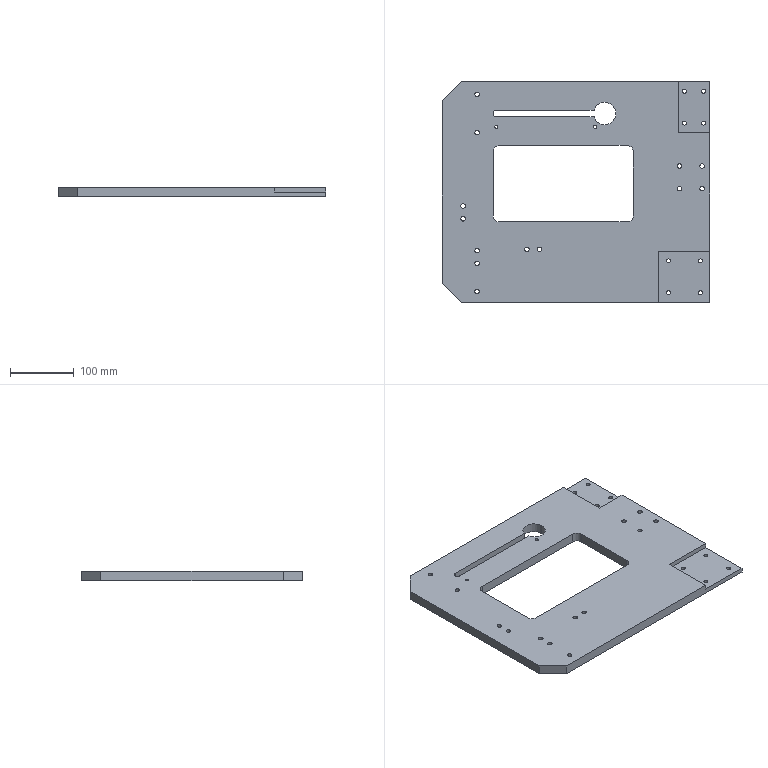Component | SolidWorks | LargeSidePlate(2)-1 | 1 solid | 105 faces | box 420 x 346 x 15 mm | volume 1641954 mm3 | cylinder 72 | plane 29 | cone 4 | commonest cylinder face diameters 7 x26 11 x18 6.2 x16 5 x4 20 x4 35 x2 10.2 x2
build123d program:
from build123d import *

# Parameters (mm, degrees)
SKETCH1_W                                            = 420
SKETCH1_H                                            = 346
BOSS_EXTRUDE1_DEPTH                                  = 15
SKETCH2_W                                            = 220
SKETCH2_H                                            = 120
CUT_EXTRUDE1_DEPTH                                   = 455.482
CUT_EXTRUDE2_DEPTH                                   = 455.482
SKETCH4_W                                            = 50
SKETCH4_H                                            = 80
CUT_EXTRUDE3_DEPTH                                   = 7.5
SKETCH5_W                                            = 80
SKETCH5_H                                            = 80
CUT_EXTRUDE4_DEPTH                                   = 7.5
SKETCH6_W                                            = 17.5
SKETCH6_H                                            = 15
F_7_0_7_DIAMETER_HOLE1_D                             = 7
F_6_2_6_2_DIAMETER_HOLE1_D                           = 6.2
F_6_2_6_2_DIAMETER_HOLE1_DEPTH                       = 15
F_5_0_5_DIAMETER_HOLE1_D                             = 5
CYLINDRICAL_COUNTERSUNK_HOLE1_FOR_M6_HEX_D           = 7
CYLINDRICAL_COUNTERSUNK_HOLE1_FOR_M6_HEX_CBORE_D     = 11
CYLINDRICAL_COUNTERSUNK_HOLE1_FOR_M6_HEX_CBORE_DEPTH = 6.5
CHAMFER1_SIZE                                        = 0.525
CHAMFER2_SIZE                                        = 30
FILLET1_R                                            = 10


with BuildPart() as part:
    # Sketch1 → Boss-Extrude1 (new body)
    with BuildSketch(Plane.XY.offset(22.5)):
        with Locations((-210, 0)):
            Rectangle(SKETCH1_W, SKETCH1_H)
    extrude(amount=-BOSS_EXTRUDE1_DEPTH)

    # Sketch2 → Cut-Extrude1 (cut, through all)
    with BuildSketch(Plane.XY.offset(22.5)):
        with Locations((-230, 13)):
            Rectangle(SKETCH2_W, SKETCH2_H)
    extrude(amount=-CUT_EXTRUDE1_DEPTH, mode=Mode.SUBTRACT)

    # Sketch3 → Cut-Extrude2 (cut, through all)
    with BuildSketch(Plane(origin=(0, 0, 7.5), x_dir=(-1, 0, 0), z_dir=(0, 0, -1))):
        with BuildLine():
            Line((335, 128.1), (181.74, 128.1))
            ThreePointArc((181.74, 128.1), (182.5, 123), (181.74, 117.9))
            Line((181.74, 117.9), (335, 117.9))
            ThreePointArc((335, 117.9), (340.1, 123), (335, 128.1))
        make_face()
    extrude(amount=-CUT_EXTRUDE2_DEPTH, mode=Mode.SUBTRACT)

    # Sketch4 → Cut-Extrude3 (cut)
    with BuildSketch(Plane.XY.offset(22.5)):
        with Locations((-25, 133)):
            Rectangle(SKETCH4_W, SKETCH4_H)
    extrude(amount=-CUT_EXTRUDE3_DEPTH, mode=Mode.SUBTRACT)

    # Sketch5 → Cut-Extrude4 (cut)
    with BuildSketch(Plane.XY.offset(22.5)):
        with Locations((-40, -133)):
            Rectangle(SKETCH5_W, SKETCH5_H)
    extrude(amount=-CUT_EXTRUDE4_DEPTH, mode=Mode.SUBTRACT)

    # Sketch6 → Cut-Revolve1 (revolve, cut)
    with BuildSketch(Plane(origin=(0, 123, 0), x_dir=(1, 0, 0), z_dir=(0, 1, 0))):
        with Locations((-156.25, -15)):
            Rectangle(SKETCH6_W, SKETCH6_H)
    revolve(axis=Axis((-165, 123, 7.5), (0, 0, 1)), mode=Mode.SUBTRACT)

    # 7.0 _7_ Diameter Hole1 (through all)
    with Locations(Plane(origin=(0, 0, 7.5), x_dir=(-1, 0, 0), z_dir=(0, 0, -1))):
        with Locations((12.322, 5.322), (47.678, 40.678), (12.322, 40.678), (47.678, 5.322)):
            Hole(F_7_0_7_DIAMETER_HOLE1_D / 2)

    # 6.2 _6.2_ Diameter Hole1
    with Locations(Plane(origin=(0, 0, 7.5), x_dir=(-1, 0, 0), z_dir=(0, 0, -1))):
        with Locations((65, -158), (65, -108), (40, 108), (40, 158), (10, 158), (10, 108), (15, -108), (15, -158)):
            Hole(F_6_2_6_2_DIAMETER_HOLE1_D / 2, depth=F_6_2_6_2_DIAMETER_HOLE1_DEPTH)

    # 5.0 _5_ Diameter Hole1 (through all)
    with Locations(Plane(origin=(0, 0, 7.5), x_dir=(-1, 0, 0), z_dir=(0, 0, -1))):
        with Locations((335, 102), (180, 102)):
            Hole(F_5_0_5_DIAMETER_HOLE1_D / 2)

    # Cylindrical Countersunk Hole1 for M6 Hex (through all)
    with Locations(Plane(origin=(0, 0, 7.5), x_dir=(-1, 0, 0), z_dir=(0, 0, -1))):
        with Locations((365, 153), (365, 93), (387, -22), (387, -42), (365, -92), (365, -112), (365, -156), (287, -90), (267, -90)):
            CounterBoreHole(CYLINDRICAL_COUNTERSUNK_HOLE1_FOR_M6_HEX_D / 2, CYLINDRICAL_COUNTERSUNK_HOLE1_FOR_M6_HEX_CBORE_D / 2, CYLINDRICAL_COUNTERSUNK_HOLE1_FOR_M6_HEX_CBORE_DEPTH)

    # Chamfer1
    chamfer1_edges = [part.edges().sort_by_distance(p)[0] for p in [
        (-182.5, 102, 7.5),
        (-337.5, 102, 7.5),
    ]]
    chamfer(chamfer1_edges, length=CHAMFER1_SIZE)

    # Chamfer2
    chamfer2_edges = [part.edges().sort_by_distance(p)[0] for p in [
        (-420, -173, 15),
        (-420, 173, 15),
    ]]
    chamfer(chamfer2_edges, length=CHAMFER2_SIZE)

    # Fillet1
    fillet1_edges = [part.edges().sort_by_distance(p)[0] for p in [
        (-340, 73, 15),
        (-120, 73, 15),
        (-120, -47, 15),
        (-340, -47, 15),
    ]]
    fillet(fillet1_edges, radius=FILLET1_R)


solid = part.part

# Placed as in the assembly
solid = solid.moved(Location((0, 438, -285), (0, 0, 0)))